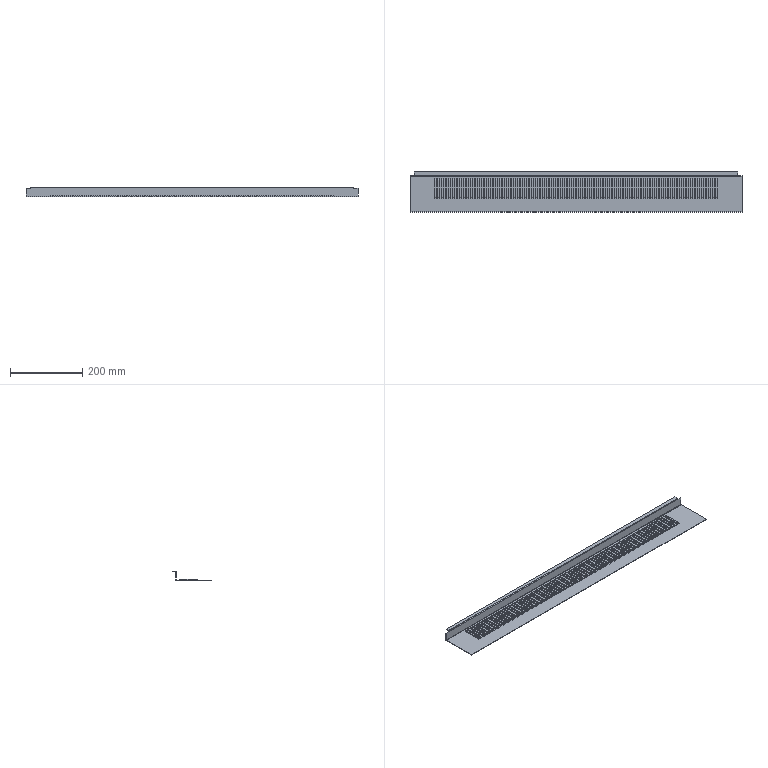Component | SolidWorks | AirFurnaceElectricalCabinet-RearLowerPlate-1 | 1 solid | 1128 faces | volume 150193 mm3 | cylinder 636 | plane 492 | commonest cylinder face diameters 6 x316 3.6 x158 8.4 x158 3.9 x2 1.5 x2